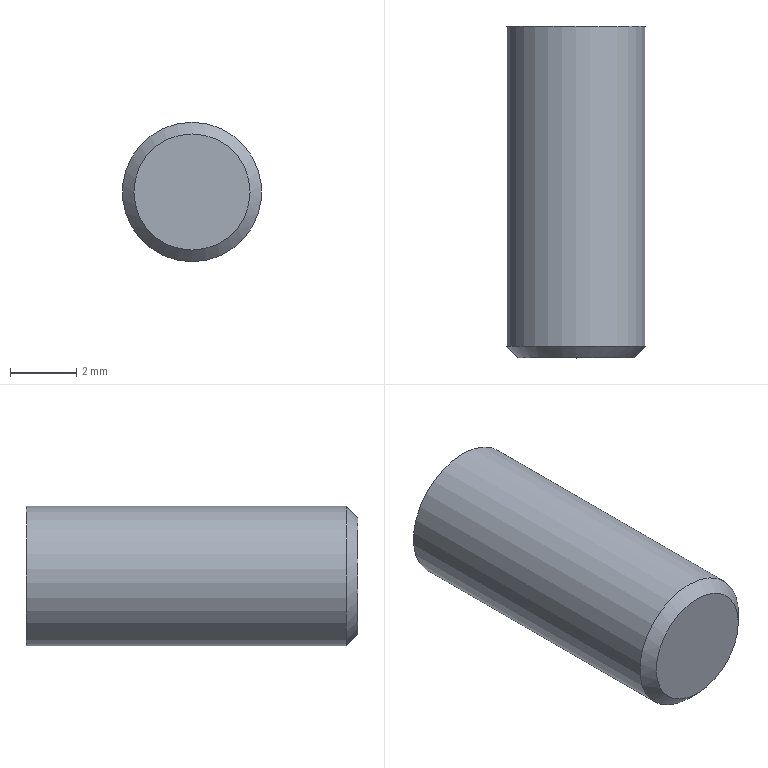Component | NX | 12_T77_2007_M5X10_FLAT_SET_SCREW | 1 solid | 11 faces | box 4.2 x 10 x 4.2 mm | volume 127 mm3 | plane 9 | cylinder 1 | cone 1 | commonest cylinder face diameters 4.2 x1
STEP:
#1=CARTESIAN_POINT('',(0.,0.,0.));
#2=DIRECTION('',(0.,0.,1.));
#3=DIRECTION('',(1.,0.,0.));
#4=AXIS2_PLACEMENT_3D('',#1,#2,#3);
#5=CARTESIAN_POINT('',(22.25,14.,74.278));
#6=VERTEX_POINT('',#5);
#7=CARTESIAN_POINT('',(22.25,14.,75.722));
#8=VERTEX_POINT('',#7);
#9=CARTESIAN_POINT('',(22.25,14.,74.278));
#10=DIRECTION('',(0.,0.,1.));
#11=VECTOR('',#10,1.);
#12=LINE('',#9,#11);
#13=CARTESIAN_POINT('',(21.,14.,75.));
#14=DIRECTION('',(0.,1.,0.));
#15=DIRECTION('',(0.,0.,-1.));
#16=AXIS2_PLACEMENT_3D('',#13,#14,#15);
#17=PLANE('',#16);
#18=CARTESIAN_POINT('',(0.7217,-1.25));
#19=DIRECTION('',(-1.,0.));
#20=VECTOR('',#19,1.);
#21=LINE('',#18,#20);
#22=(GEOMETRIC_REPRESENTATION_CONTEXT(2)PARAMETRIC_REPRESENTATION_CONTEXT()REPRESENTATION_CONTEXT('',''));
#23=DEFINITIONAL_REPRESENTATION('',(#21),#22);
#24=PCURVE('',#17,#23);
#25=CARTESIAN_POINT('',(22.25,12.,74.278));
#26=DIRECTION('',(-1.,0.,0.));
#27=DIRECTION('',(0.,0.,1.));
#28=AXIS2_PLACEMENT_3D('',#25,#26,#27);
#29=PLANE('',#28);
#30=CARTESIAN_POINT('',(0.,2.));
#31=DIRECTION('',(1.,0.));
#32=VECTOR('',#31,1.);
#33=LINE('',#30,#32);
#34=(GEOMETRIC_REPRESENTATION_CONTEXT(2)PARAMETRIC_REPRESENTATION_CONTEXT()REPRESENTATION_CONTEXT('',''));
#35=DEFINITIONAL_REPRESENTATION('',(#33),#34);
#36=PCURVE('',#29,#35);
#37=SURFACE_CURVE('',#12,(#24,#36),.PCURVE_S1.);
#38=EDGE_CURVE('',#6,#8,#37,.T.);
#39=ORIENTED_EDGE('',*,*,#38,.T.);
#40=CARTESIAN_POINT('',(21.,14.,76.443));
#41=VERTEX_POINT('',#40);
#42=CARTESIAN_POINT('',(22.25,14.,75.722));
#43=DIRECTION('',(-0.866,0.,0.5));
#44=VECTOR('',#43,1.);
#45=LINE('',#42,#44);
#46=CARTESIAN_POINT('',(-0.7217,-1.25));
#47=DIRECTION('',(-0.5,0.866));
#48=VECTOR('',#47,1.);
#49=LINE('',#46,#48);
#50=(GEOMETRIC_REPRESENTATION_CONTEXT(2)PARAMETRIC_REPRESENTATION_CONTEXT()REPRESENTATION_CONTEXT('',''));
#51=DEFINITIONAL_REPRESENTATION('',(#49),#50);
#52=PCURVE('',#17,#51);
#53=CARTESIAN_POINT('',(22.25,12.,75.722));
#54=DIRECTION('',(-0.5,0.,-0.866));
#55=DIRECTION('',(-0.866,0.,0.5));
#56=AXIS2_PLACEMENT_3D('',#53,#54,#55);
#57=PLANE('',#56);
#58=CARTESIAN_POINT('',(0.,2.));
#59=DIRECTION('',(1.,0.));
#60=VECTOR('',#59,1.);
#61=LINE('',#58,#60);
#62=(GEOMETRIC_REPRESENTATION_CONTEXT(2)PARAMETRIC_REPRESENTATION_CONTEXT()REPRESENTATION_CONTEXT('',''));
#63=DEFINITIONAL_REPRESENTATION('',(#61),#62);
#64=PCURVE('',#57,#63);
#65=SURFACE_CURVE('',#45,(#52,#64),.PCURVE_S1.);
#66=EDGE_CURVE('',#8,#41,#65,.T.);
#67=ORIENTED_EDGE('',*,*,#66,.T.);
#68=CARTESIAN_POINT('',(19.75,14.,75.722));
#69=VERTEX_POINT('',#68);
#70=CARTESIAN_POINT('',(21.,14.,76.443));
#71=DIRECTION('',(-0.866,0.,-0.5));
#72=VECTOR('',#71,1.);
#73=LINE('',#70,#72);
#74=CARTESIAN_POINT('',(-1.443,0.));
#75=DIRECTION('',(0.5,0.866));
#76=VECTOR('',#75,1.);
#77=LINE('',#74,#76);
#78=(GEOMETRIC_REPRESENTATION_CONTEXT(2)PARAMETRIC_REPRESENTATION_CONTEXT()REPRESENTATION_CONTEXT('',''));
#79=DEFINITIONAL_REPRESENTATION('',(#77),#78);
#80=PCURVE('',#17,#79);
#81=CARTESIAN_POINT('',(21.,12.,76.443));
#82=DIRECTION('',(0.5,0.,-0.866));
#83=DIRECTION('',(-0.866,0.,-0.5));
#84=AXIS2_PLACEMENT_3D('',#81,#82,#83);
#85=PLANE('',#84);
#86=CARTESIAN_POINT('',(0.,2.));
#87=DIRECTION('',(1.,0.));
#88=VECTOR('',#87,1.);
#89=LINE('',#86,#88);
#90=(GEOMETRIC_REPRESENTATION_CONTEXT(2)PARAMETRIC_REPRESENTATION_CONTEXT()REPRESENTATION_CONTEXT('',''));
#91=DEFINITIONAL_REPRESENTATION('',(#89),#90);
#92=PCURVE('',#85,#91);
#93=SURFACE_CURVE('',#73,(#80,#92),.PCURVE_S1.);
#94=EDGE_CURVE('',#41,#69,#93,.T.);
#95=ORIENTED_EDGE('',*,*,#94,.T.);
#96=CARTESIAN_POINT('',(19.75,14.,74.278));
#97=VERTEX_POINT('',#96);
#98=CARTESIAN_POINT('',(19.75,14.,75.722));
#99=DIRECTION('',(0.,0.,-1.));
#100=VECTOR('',#99,1.);
#101=LINE('',#98,#100);
#102=CARTESIAN_POINT('',(-0.7217,1.25));
#103=DIRECTION('',(1.,0.));
#104=VECTOR('',#103,1.);
#105=LINE('',#102,#104);
#106=(GEOMETRIC_REPRESENTATION_CONTEXT(2)PARAMETRIC_REPRESENTATION_CONTEXT()REPRESENTATION_CONTEXT('',''));
#107=DEFINITIONAL_REPRESENTATION('',(#105),#106);
#108=PCURVE('',#17,#107);
#109=CARTESIAN_POINT('',(19.75,12.,75.722));
#110=DIRECTION('',(1.,0.,0.));
#111=DIRECTION('',(0.,0.,-1.));
#112=AXIS2_PLACEMENT_3D('',#109,#110,#111);
#113=PLANE('',#112);
#114=CARTESIAN_POINT('',(0.,2.));
#115=DIRECTION('',(1.,0.));
#116=VECTOR('',#115,1.);
#117=LINE('',#114,#116);
#118=(GEOMETRIC_REPRESENTATION_CONTEXT(2)PARAMETRIC_REPRESENTATION_CONTEXT()REPRESENTATION_CONTEXT('',''));
#119=DEFINITIONAL_REPRESENTATION('',(#117),#118);
#120=PCURVE('',#113,#119);
#121=SURFACE_CURVE('',#101,(#108,#120),.PCURVE_S1.);
#122=EDGE_CURVE('',#69,#97,#121,.T.);
#123=ORIENTED_EDGE('',*,*,#122,.T.);
#124=CARTESIAN_POINT('',(21.,14.,73.557));
#125=VERTEX_POINT('',#124);
#126=CARTESIAN_POINT('',(19.75,14.,74.278));
#127=DIRECTION('',(0.866,-0.,-0.5));
#128=VECTOR('',#127,1.);
#129=LINE('',#126,#128);
#130=CARTESIAN_POINT('',(0.7217,1.25));
#131=DIRECTION('',(0.5,-0.866));
#132=VECTOR('',#131,1.);
#133=LINE('',#130,#132);
#134=(GEOMETRIC_REPRESENTATION_CONTEXT(2)PARAMETRIC_REPRESENTATION_CONTEXT()REPRESENTATION_CONTEXT('',''));
#135=DEFINITIONAL_REPRESENTATION('',(#133),#134);
#136=PCURVE('',#17,#135);
#137=CARTESIAN_POINT('',(19.75,12.,74.278));
#138=DIRECTION('',(0.5,0.,0.866));
#139=DIRECTION('',(0.866,0.,-0.5));
#140=AXIS2_PLACEMENT_3D('',#137,#138,#139);
#141=PLANE('',#140);
#142=CARTESIAN_POINT('',(0.,2.));
#143=DIRECTION('',(1.,-0.));
#144=VECTOR('',#143,1.);
#145=LINE('',#142,#144);
#146=(GEOMETRIC_REPRESENTATION_CONTEXT(2)PARAMETRIC_REPRESENTATION_CONTEXT()REPRESENTATION_CONTEXT('',''));
#147=DEFINITIONAL_REPRESENTATION('',(#145),#146);
#148=PCURVE('',#141,#147);
#149=SURFACE_CURVE('',#129,(#136,#148),.PCURVE_S1.);
#150=EDGE_CURVE('',#97,#125,#149,.T.);
#151=ORIENTED_EDGE('',*,*,#150,.T.);
#152=CARTESIAN_POINT('',(21.,14.,73.557));
#153=DIRECTION('',(0.866,-0.,0.5));
#154=VECTOR('',#153,1.);
#155=LINE('',#152,#154);
#156=CARTESIAN_POINT('',(1.443,0.));
#157=DIRECTION('',(-0.5,-0.866));
#158=VECTOR('',#157,1.);
#159=LINE('',#156,#158);
#160=(GEOMETRIC_REPRESENTATION_CONTEXT(2)PARAMETRIC_REPRESENTATION_CONTEXT()REPRESENTATION_CONTEXT('',''));
#161=DEFINITIONAL_REPRESENTATION('',(#159),#160);
#162=PCURVE('',#17,#161);
#163=CARTESIAN_POINT('',(21.,12.,73.557));
#164=DIRECTION('',(-0.5,0.,0.866));
#165=DIRECTION('',(0.866,0.,0.5));
#166=AXIS2_PLACEMENT_3D('',#163,#164,#165);
#167=PLANE('',#166);
#168=CARTESIAN_POINT('',(0.,2.));
#169=DIRECTION('',(1.,-0.));
#170=VECTOR('',#169,1.);
#171=LINE('',#168,#170);
#172=(GEOMETRIC_REPRESENTATION_CONTEXT(2)PARAMETRIC_REPRESENTATION_CONTEXT()REPRESENTATION_CONTEXT('',''));
#173=DEFINITIONAL_REPRESENTATION('',(#171),#172);
#174=PCURVE('',#167,#173);
#175=SURFACE_CURVE('',#155,(#162,#174),.PCURVE_S1.);
#176=EDGE_CURVE('',#125,#6,#175,.T.);
#177=ORIENTED_EDGE('',*,*,#176,.T.);
#178=EDGE_LOOP('',(#39,#67,#95,#123,#151,#177));
#179=FACE_BOUND('',#178,.T.);
#180=CARTESIAN_POINT('',(21.,14.,77.1));
#181=VERTEX_POINT('',#180);
#182=CARTESIAN_POINT('',(21.,14.,75.));
#183=DIRECTION('',(0.,1.,0.));
#184=DIRECTION('',(0.,-0.,1.));
#185=AXIS2_PLACEMENT_3D('',#182,#183,#184);
#186=CIRCLE('',#185,2.1);
#187=CARTESIAN_POINT('',(0.,0.));
#188=DIRECTION('',(-1.,0.));
#189=AXIS2_PLACEMENT_2D('',#187,#188);
#190=CIRCLE('',#189,2.1);
#191=(GEOMETRIC_REPRESENTATION_CONTEXT(2)PARAMETRIC_REPRESENTATION_CONTEXT()REPRESENTATION_CONTEXT('',''));
#192=DEFINITIONAL_REPRESENTATION('',(#190),#191);
#193=PCURVE('',#17,#192);
#194=CARTESIAN_POINT('',(21.,15.5,75.));
#195=DIRECTION('',(0.,-1.,0.));
#196=DIRECTION('',(0.,0.,-1.));
#197=AXIS2_PLACEMENT_3D('',#194,#195,#196);
#198=CYLINDRICAL_SURFACE('',#197,2.1);
#199=CARTESIAN_POINT('',(9.425,1.5));
#200=DIRECTION('',(-1.,0.));
#201=VECTOR('',#200,1.);
#202=LINE('',#199,#201);
#203=(GEOMETRIC_REPRESENTATION_CONTEXT(2)PARAMETRIC_REPRESENTATION_CONTEXT()REPRESENTATION_CONTEXT('',''));
#204=DEFINITIONAL_REPRESENTATION('',(#202),#203);
#205=PCURVE('',#198,#204);
#206=SURFACE_CURVE('',#186,(#193,#205),.PCURVE_S1.);
#207=EDGE_CURVE('',#181,#181,#206,.T.);
#208=ORIENTED_EDGE('',*,*,#207,.T.);
#209=EDGE_LOOP('',(#208));
#210=FACE_BOUND('',#209,.T.);
#211=ADVANCED_FACE('',(#179,#210),#17,.T.);
#212=ORIENTED_EDGE('',*,*,#66,.F.);
#213=CARTESIAN_POINT('',(22.25,12.,75.722));
#214=VERTEX_POINT('',#213);
#215=CARTESIAN_POINT('',(22.25,12.,75.722));
#216=DIRECTION('',(0.,1.,0.));
#217=VECTOR('',#216,1.);
#218=LINE('',#215,#217);
#219=CARTESIAN_POINT('',(0.,0.));
#220=DIRECTION('',(0.,1.));
#221=VECTOR('',#220,1.);
#222=LINE('',#219,#221);
#223=(GEOMETRIC_REPRESENTATION_CONTEXT(2)PARAMETRIC_REPRESENTATION_CONTEXT()REPRESENTATION_CONTEXT('',''));
#224=DEFINITIONAL_REPRESENTATION('',(#222),#223);
#225=PCURVE('',#57,#224);
#226=CARTESIAN_POINT('',(1.443,0.));
#227=DIRECTION('',(0.,1.));
#228=VECTOR('',#227,1.);
#229=LINE('',#226,#228);
#230=(GEOMETRIC_REPRESENTATION_CONTEXT(2)PARAMETRIC_REPRESENTATION_CONTEXT()REPRESENTATION_CONTEXT('',''));
#231=DEFINITIONAL_REPRESENTATION('',(#229),#230);
#232=PCURVE('',#29,#231);
#233=SURFACE_CURVE('',#218,(#225,#232),.PCURVE_S1.);
#234=EDGE_CURVE('',#214,#8,#233,.T.);
#235=ORIENTED_EDGE('',*,*,#234,.F.);
#236=CARTESIAN_POINT('',(21.,12.,76.443));
#237=VERTEX_POINT('',#236);
#238=CARTESIAN_POINT('',(22.25,12.,75.722));
#239=DIRECTION('',(-0.866,0.,0.5));
#240=VECTOR('',#239,1.);
#241=LINE('',#238,#240);
#242=CARTESIAN_POINT('',(0.,0.));
#243=DIRECTION('',(1.,0.));
#244=VECTOR('',#243,1.);
#245=LINE('',#242,#244);
#246=(GEOMETRIC_REPRESENTATION_CONTEXT(2)PARAMETRIC_REPRESENTATION_CONTEXT()REPRESENTATION_CONTEXT('',''));
#247=DEFINITIONAL_REPRESENTATION('',(#245),#246);
#248=PCURVE('',#57,#247);
#249=CARTESIAN_POINT('',(21.,12.,75.));
#250=DIRECTION('',(-0.,-1.,0.));
#251=DIRECTION('',(-1.,0.,0.));
#252=AXIS2_PLACEMENT_3D('',#249,#250,#251);
#253=PLANE('',#252);
#254=CARTESIAN_POINT('',(-1.25,-0.7217));
#255=DIRECTION('',(0.866,-0.5));
#256=VECTOR('',#255,1.);
#257=LINE('',#254,#256);
#258=(GEOMETRIC_REPRESENTATION_CONTEXT(2)PARAMETRIC_REPRESENTATION_CONTEXT()REPRESENTATION_CONTEXT('',''));
#259=DEFINITIONAL_REPRESENTATION('',(#257),#258);
#260=PCURVE('',#253,#259);
#261=SURFACE_CURVE('',#241,(#248,#260),.PCURVE_S1.);
#262=EDGE_CURVE('',#214,#237,#261,.T.);
#263=ORIENTED_EDGE('',*,*,#262,.T.);
#264=CARTESIAN_POINT('',(21.,12.,76.443));
#265=DIRECTION('',(0.,1.,0.));
#266=VECTOR('',#265,1.);
#267=LINE('',#264,#266);
#268=CARTESIAN_POINT('',(1.443,0.));
#269=DIRECTION('',(0.,1.));
#270=VECTOR('',#269,1.);
#271=LINE('',#268,#270);
#272=(GEOMETRIC_REPRESENTATION_CONTEXT(2)PARAMETRIC_REPRESENTATION_CONTEXT()REPRESENTATION_CONTEXT('',''));
#273=DEFINITIONAL_REPRESENTATION('',(#271),#272);
#274=PCURVE('',#57,#273);
#275=CARTESIAN_POINT('',(0.,0.));
#276=DIRECTION('',(0.,1.));
#277=VECTOR('',#276,1.);
#278=LINE('',#275,#277);
#279=(GEOMETRIC_REPRESENTATION_CONTEXT(2)PARAMETRIC_REPRESENTATION_CONTEXT()REPRESENTATION_CONTEXT('',''));
#280=DEFINITIONAL_REPRESENTATION('',(#278),#279);
#281=PCURVE('',#85,#280);
#282=SURFACE_CURVE('',#267,(#274,#281),.PCURVE_S1.);
#283=EDGE_CURVE('',#237,#41,#282,.T.);
#284=ORIENTED_EDGE('',*,*,#283,.T.);
#285=EDGE_LOOP('',(#212,#235,#263,#284));
#286=FACE_BOUND('',#285,.T.);
#287=ADVANCED_FACE('',(#286),#57,.T.);
#288=ORIENTED_EDGE('',*,*,#94,.F.);
#289=ORIENTED_EDGE('',*,*,#283,.F.);
#290=CARTESIAN_POINT('',(19.75,12.,75.722));
#291=VERTEX_POINT('',#290);
#292=CARTESIAN_POINT('',(21.,12.,76.443));
#293=DIRECTION('',(-0.866,0.,-0.5));
#294=VECTOR('',#293,1.);
#295=LINE('',#292,#294);
#296=CARTESIAN_POINT('',(0.,0.));
#297=DIRECTION('',(1.,0.));
#298=VECTOR('',#297,1.);
#299=LINE('',#296,#298);
#300=(GEOMETRIC_REPRESENTATION_CONTEXT(2)PARAMETRIC_REPRESENTATION_CONTEXT()REPRESENTATION_CONTEXT('',''));
#301=DEFINITIONAL_REPRESENTATION('',(#299),#300);
#302=PCURVE('',#85,#301);
#303=CARTESIAN_POINT('',(0.,-1.443));
#304=DIRECTION('',(0.866,0.5));
#305=VECTOR('',#304,1.);
#306=LINE('',#303,#305);
#307=(GEOMETRIC_REPRESENTATION_CONTEXT(2)PARAMETRIC_REPRESENTATION_CONTEXT()REPRESENTATION_CONTEXT('',''));
#308=DEFINITIONAL_REPRESENTATION('',(#306),#307);
#309=PCURVE('',#253,#308);
#310=SURFACE_CURVE('',#295,(#302,#309),.PCURVE_S1.);
#311=EDGE_CURVE('',#237,#291,#310,.T.);
#312=ORIENTED_EDGE('',*,*,#311,.T.);
#313=CARTESIAN_POINT('',(19.75,12.,75.722));
#314=DIRECTION('',(0.,1.,0.));
#315=VECTOR('',#314,1.);
#316=LINE('',#313,#315);
#317=CARTESIAN_POINT('',(1.443,0.));
#318=DIRECTION('',(0.,1.));
#319=VECTOR('',#318,1.);
#320=LINE('',#317,#319);
#321=(GEOMETRIC_REPRESENTATION_CONTEXT(2)PARAMETRIC_REPRESENTATION_CONTEXT()REPRESENTATION_CONTEXT('',''));
#322=DEFINITIONAL_REPRESENTATION('',(#320),#321);
#323=PCURVE('',#85,#322);
#324=CARTESIAN_POINT('',(0.,0.));
#325=DIRECTION('',(0.,1.));
#326=VECTOR('',#325,1.);
#327=LINE('',#324,#326);
#328=(GEOMETRIC_REPRESENTATION_CONTEXT(2)PARAMETRIC_REPRESENTATION_CONTEXT()REPRESENTATION_CONTEXT('',''));
#329=DEFINITIONAL_REPRESENTATION('',(#327),#328);
#330=PCURVE('',#113,#329);
#331=SURFACE_CURVE('',#316,(#323,#330),.PCURVE_S1.);
#332=EDGE_CURVE('',#291,#69,#331,.T.);
#333=ORIENTED_EDGE('',*,*,#332,.T.);
#334=EDGE_LOOP('',(#288,#289,#312,#333));
#335=FACE_BOUND('',#334,.T.);
#336=ADVANCED_FACE('',(#335),#85,.T.);
#337=ORIENTED_EDGE('',*,*,#122,.F.);
#338=ORIENTED_EDGE('',*,*,#332,.F.);
#339=CARTESIAN_POINT('',(19.75,12.,74.278));
#340=VERTEX_POINT('',#339);
#341=CARTESIAN_POINT('',(19.75,12.,75.722));
#342=DIRECTION('',(0.,0.,-1.));
#343=VECTOR('',#342,1.);
#344=LINE('',#341,#343);
#345=CARTESIAN_POINT('',(0.,0.));
#346=DIRECTION('',(1.,0.));
#347=VECTOR('',#346,1.);
#348=LINE('',#345,#347);
#349=(GEOMETRIC_REPRESENTATION_CONTEXT(2)PARAMETRIC_REPRESENTATION_CONTEXT()REPRESENTATION_CONTEXT('',''));
#350=DEFINITIONAL_REPRESENTATION('',(#348),#349);
#351=PCURVE('',#113,#350);
#352=CARTESIAN_POINT('',(1.25,-0.7217));
#353=DIRECTION('',(0.,1.));
#354=VECTOR('',#353,1.);
#355=LINE('',#352,#354);
#356=(GEOMETRIC_REPRESENTATION_CONTEXT(2)PARAMETRIC_REPRESENTATION_CONTEXT()REPRESENTATION_CONTEXT('',''));
#357=DEFINITIONAL_REPRESENTATION('',(#355),#356);
#358=PCURVE('',#253,#357);
#359=SURFACE_CURVE('',#344,(#351,#358),.PCURVE_S1.);
#360=EDGE_CURVE('',#291,#340,#359,.T.);
#361=ORIENTED_EDGE('',*,*,#360,.T.);
#362=CARTESIAN_POINT('',(19.75,12.,74.278));
#363=DIRECTION('',(0.,1.,0.));
#364=VECTOR('',#363,1.);
#365=LINE('',#362,#364);
#366=CARTESIAN_POINT('',(1.443,0.));
#367=DIRECTION('',(0.,1.));
#368=VECTOR('',#367,1.);
#369=LINE('',#366,#368);
#370=(GEOMETRIC_REPRESENTATION_CONTEXT(2)PARAMETRIC_REPRESENTATION_CONTEXT()REPRESENTATION_CONTEXT('',''));
#371=DEFINITIONAL_REPRESENTATION('',(#369),#370);
#372=PCURVE('',#113,#371);
#373=CARTESIAN_POINT('',(0.,0.));
#374=DIRECTION('',(0.,1.));
#375=VECTOR('',#374,1.);
#376=LINE('',#373,#375);
#377=(GEOMETRIC_REPRESENTATION_CONTEXT(2)PARAMETRIC_REPRESENTATION_CONTEXT()REPRESENTATION_CONTEXT('',''));
#378=DEFINITIONAL_REPRESENTATION('',(#376),#377);
#379=PCURVE('',#141,#378);
#380=SURFACE_CURVE('',#365,(#372,#379),.PCURVE_S1.);
#381=EDGE_CURVE('',#340,#97,#380,.T.);
#382=ORIENTED_EDGE('',*,*,#381,.T.);
#383=EDGE_LOOP('',(#337,#338,#361,#382));
#384=FACE_BOUND('',#383,.T.);
#385=ADVANCED_FACE('',(#384),#113,.T.);
#386=ORIENTED_EDGE('',*,*,#150,.F.);
#387=ORIENTED_EDGE('',*,*,#381,.F.);
#388=CARTESIAN_POINT('',(21.,12.,73.557));
#389=VERTEX_POINT('',#388);
#390=CARTESIAN_POINT('',(19.75,12.,74.278));
#391=DIRECTION('',(0.866,-0.,-0.5));
#392=VECTOR('',#391,1.);
#393=LINE('',#390,#392);
#394=CARTESIAN_POINT('',(0.,0.));
#395=DIRECTION('',(1.,-0.));
#396=VECTOR('',#395,1.);
#397=LINE('',#394,#396);
#398=(GEOMETRIC_REPRESENTATION_CONTEXT(2)PARAMETRIC_REPRESENTATION_CONTEXT()REPRESENTATION_CONTEXT('',''));
#399=DEFINITIONAL_REPRESENTATION('',(#397),#398);
#400=PCURVE('',#141,#399);
#401=CARTESIAN_POINT('',(1.25,0.7217));
#402=DIRECTION('',(-0.866,0.5));
#403=VECTOR('',#402,1.);
#404=LINE('',#401,#403);
#405=(GEOMETRIC_REPRESENTATION_CONTEXT(2)PARAMETRIC_REPRESENTATION_CONTEXT()REPRESENTATION_CONTEXT('',''));
#406=DEFINITIONAL_REPRESENTATION('',(#404),#405);
#407=PCURVE('',#253,#406);
#408=SURFACE_CURVE('',#393,(#400,#407),.PCURVE_S1.);
#409=EDGE_CURVE('',#340,#389,#408,.T.);
#410=ORIENTED_EDGE('',*,*,#409,.T.);
#411=CARTESIAN_POINT('',(21.,12.,73.557));
#412=DIRECTION('',(0.,1.,0.));
#413=VECTOR('',#412,1.);
#414=LINE('',#411,#413);
#415=CARTESIAN_POINT('',(1.443,0.));
#416=DIRECTION('',(0.,1.));
#417=VECTOR('',#416,1.);
#418=LINE('',#415,#417);
#419=(GEOMETRIC_REPRESENTATION_CONTEXT(2)PARAMETRIC_REPRESENTATION_CONTEXT()REPRESENTATION_CONTEXT('',''));
#420=DEFINITIONAL_REPRESENTATION('',(#418),#419);
#421=PCURVE('',#141,#420);
#422=CARTESIAN_POINT('',(0.,0.));
#423=DIRECTION('',(0.,1.));
#424=VECTOR('',#423,1.);
#425=LINE('',#422,#424);
#426=(GEOMETRIC_REPRESENTATION_CONTEXT(2)PARAMETRIC_REPRESENTATION_CONTEXT()REPRESENTATION_CONTEXT('',''));
#427=DEFINITIONAL_REPRESENTATION('',(#425),#426);
#428=PCURVE('',#167,#427);
#429=SURFACE_CURVE('',#414,(#421,#428),.PCURVE_S1.);
#430=EDGE_CURVE('',#389,#125,#429,.T.);
#431=ORIENTED_EDGE('',*,*,#430,.T.);
#432=EDGE_LOOP('',(#386,#387,#410,#431));
#433=FACE_BOUND('',#432,.T.);
#434=ADVANCED_FACE('',(#433),#141,.T.);
#435=ORIENTED_EDGE('',*,*,#176,.F.);
#436=ORIENTED_EDGE('',*,*,#430,.F.);
#437=CARTESIAN_POINT('',(22.25,12.,74.278));
#438=VERTEX_POINT('',#437);
#439=CARTESIAN_POINT('',(21.,12.,73.557));
#440=DIRECTION('',(0.866,-0.,0.5));
#441=VECTOR('',#440,1.);
#442=LINE('',#439,#441);
#443=CARTESIAN_POINT('',(0.,0.));
#444=DIRECTION('',(1.,-0.));
#445=VECTOR('',#444,1.);
#446=LINE('',#443,#445);
#447=(GEOMETRIC_REPRESENTATION_CONTEXT(2)PARAMETRIC_REPRESENTATION_CONTEXT()REPRESENTATION_CONTEXT('',''));
#448=DEFINITIONAL_REPRESENTATION('',(#446),#447);
#449=PCURVE('',#167,#448);
#450=CARTESIAN_POINT('',(0.,1.443));
#451=DIRECTION('',(-0.866,-0.5));
#452=VECTOR('',#451,1.);
#453=LINE('',#450,#452);
#454=(GEOMETRIC_REPRESENTATION_CONTEXT(2)PARAMETRIC_REPRESENTATION_CONTEXT()REPRESENTATION_CONTEXT('',''));
#455=DEFINITIONAL_REPRESENTATION('',(#453),#454);
#456=PCURVE('',#253,#455);
#457=SURFACE_CURVE('',#442,(#449,#456),.PCURVE_S1.);
#458=EDGE_CURVE('',#389,#438,#457,.T.);
#459=ORIENTED_EDGE('',*,*,#458,.T.);
#460=CARTESIAN_POINT('',(22.25,12.,74.278));
#461=DIRECTION('',(0.,1.,0.));
#462=VECTOR('',#461,1.);
#463=LINE('',#460,#462);
#464=CARTESIAN_POINT('',(1.443,0.));
#465=DIRECTION('',(0.,1.));
#466=VECTOR('',#465,1.);
#467=LINE('',#464,#466);
#468=(GEOMETRIC_REPRESENTATION_CONTEXT(2)PARAMETRIC_REPRESENTATION_CONTEXT()REPRESENTATION_CONTEXT('',''));
#469=DEFINITIONAL_REPRESENTATION('',(#467),#468);
#470=PCURVE('',#167,#469);
#471=CARTESIAN_POINT('',(0.,0.));
#472=DIRECTION('',(0.,1.));
#473=VECTOR('',#472,1.);
#474=LINE('',#471,#473);
#475=(GEOMETRIC_REPRESENTATION_CONTEXT(2)PARAMETRIC_REPRESENTATION_CONTEXT()REPRESENTATION_CONTEXT('',''));
#476=DEFINITIONAL_REPRESENTATION('',(#474),#475);
#477=PCURVE('',#29,#476);
#478=SURFACE_CURVE('',#463,(#470,#477),.PCURVE_S1.);
#479=EDGE_CURVE('',#438,#6,#478,.T.);
#480=ORIENTED_EDGE('',*,*,#479,.T.);
#481=EDGE_LOOP('',(#435,#436,#459,#480));
#482=FACE_BOUND('',#481,.T.);
#483=ADVANCED_FACE('',(#482),#167,.T.);
#484=ORIENTED_EDGE('',*,*,#38,.F.);
#485=ORIENTED_EDGE('',*,*,#479,.F.);
#486=CARTESIAN_POINT('',(22.25,12.,74.278));
#487=DIRECTION('',(0.,0.,1.));
#488=VECTOR('',#487,1.);
#489=LINE('',#486,#488);
#490=CARTESIAN_POINT('',(0.,0.));
#491=DIRECTION('',(1.,0.));
#492=VECTOR('',#491,1.);
#493=LINE('',#490,#492);
#494=(GEOMETRIC_REPRESENTATION_CONTEXT(2)PARAMETRIC_REPRESENTATION_CONTEXT()REPRESENTATION_CONTEXT('',''));
#495=DEFINITIONAL_REPRESENTATION('',(#493),#494);
#496=PCURVE('',#29,#495);
#497=CARTESIAN_POINT('',(-1.25,0.7217));
#498=DIRECTION('',(0.,-1.));
#499=VECTOR('',#498,1.);
#500=LINE('',#497,#499);
#501=(GEOMETRIC_REPRESENTATION_CONTEXT(2)PARAMETRIC_REPRESENTATION_CONTEXT()REPRESENTATION_CONTEXT('',''));
#502=DEFINITIONAL_REPRESENTATION('',(#500),#501);
#503=PCURVE('',#253,#502);
#504=SURFACE_CURVE('',#489,(#496,#503),.PCURVE_S1.);
#505=EDGE_CURVE('',#438,#214,#504,.T.);
#506=ORIENTED_EDGE('',*,*,#505,.T.);
#507=ORIENTED_EDGE('',*,*,#234,.T.);
#508=EDGE_LOOP('',(#484,#485,#506,#507));
#509=FACE_BOUND('',#508,.T.);
#510=ADVANCED_FACE('',(#509),#29,.T.);
#511=ORIENTED_EDGE('',*,*,#262,.F.);
#512=ORIENTED_EDGE('',*,*,#505,.F.);
#513=ORIENTED_EDGE('',*,*,#458,.F.);
#514=ORIENTED_EDGE('',*,*,#409,.F.);
#515=ORIENTED_EDGE('',*,*,#360,.F.);
#516=ORIENTED_EDGE('',*,*,#311,.F.);
#517=EDGE_LOOP('',(#511,#512,#513,#514,#515,#516));
#518=FACE_BOUND('',#517,.T.);
#519=ADVANCED_FACE('',(#518),#253,.F.);
#520=ORIENTED_EDGE('',*,*,#207,.F.);
#521=CARTESIAN_POINT('',(21.,4.35,77.1));
#522=VERTEX_POINT('',#521);
#523=CARTESIAN_POINT('',(21.,14.,77.1));
#524=CARTESIAN_POINT('',(21.,4.35,77.1));
#525=B_SPLINE_CURVE_WITH_KNOTS('',1,(#523,#524),.UNSPECIFIED.,.F.,.F.,(2,2),(1.5,11.15),.PIECEWISE_BEZIER_KNOTS.);
#526=CARTESIAN_POINT('',(9.425,0.));
#527=DIRECTION('',(0.,1.));
#528=VECTOR('',#527,1.);
#529=LINE('',#526,#528);
#530=(GEOMETRIC_REPRESENTATION_CONTEXT(2)PARAMETRIC_REPRESENTATION_CONTEXT()REPRESENTATION_CONTEXT('',''));
#531=DEFINITIONAL_REPRESENTATION('',(#529),#530);
#532=PCURVE('',#198,#531);
#533=CARTESIAN_POINT('',(3.142,0.));
#534=DIRECTION('',(0.,1.));
#535=VECTOR('',#534,1.);
#536=LINE('',#533,#535);
#537=(GEOMETRIC_REPRESENTATION_CONTEXT(2)PARAMETRIC_REPRESENTATION_CONTEXT()REPRESENTATION_CONTEXT('',''));
#538=DEFINITIONAL_REPRESENTATION('',(#536),#537);
#539=PCURVE('',#198,#538);
#540=SEAM_CURVE('',#525,(#532,#539),.PCURVE_S1.);
#541=EDGE_CURVE('',#181,#522,#540,.T.);
#542=ORIENTED_EDGE('',*,*,#541,.T.);
#543=CARTESIAN_POINT('',(21.,4.35,75.));
#544=DIRECTION('',(0.,-1.,-0.));
#545=DIRECTION('',(0.,-0.,1.));
#546=AXIS2_PLACEMENT_3D('',#543,#544,#545);
#547=CIRCLE('',#546,2.1);
#548=CARTESIAN_POINT('',(3.142,11.15));
#549=DIRECTION('',(1.,0.));
#550=VECTOR('',#549,1.);
#551=LINE('',#548,#550);
#552=(GEOMETRIC_REPRESENTATION_CONTEXT(2)PARAMETRIC_REPRESENTATION_CONTEXT()REPRESENTATION_CONTEXT('',''));
#553=DEFINITIONAL_REPRESENTATION('',(#551),#552);
#554=PCURVE('',#198,#553);
#555=CARTESIAN_POINT('',(21.,4.75,75.));
#556=DIRECTION('',(0.,1.,0.));
#557=DIRECTION('',(0.,0.,-1.));
#558=AXIS2_PLACEMENT_3D('',#555,#556,#557);
#559=CONICAL_SURFACE('',#558,2.5,0.7854);
#560=CARTESIAN_POINT('',(9.425,-0.4));
#561=DIRECTION('',(-1.,0.));
#562=VECTOR('',#561,1.);
#563=LINE('',#560,#562);
#564=(GEOMETRIC_REPRESENTATION_CONTEXT(2)PARAMETRIC_REPRESENTATION_CONTEXT()REPRESENTATION_CONTEXT('',''));
#565=DEFINITIONAL_REPRESENTATION('',(#563),#564);
#566=PCURVE('',#559,#565);
#567=SURFACE_CURVE('',#547,(#554,#566),.PCURVE_S1.);
#568=EDGE_CURVE('',#522,#522,#567,.T.);
#569=ORIENTED_EDGE('',*,*,#568,.F.);
#570=ORIENTED_EDGE('',*,*,#541,.F.);
#571=EDGE_LOOP('',(#520,#542,#569,#570));
#572=FACE_BOUND('',#571,.T.);
#573=ADVANCED_FACE('',(#572),#198,.T.);
#574=CARTESIAN_POINT('',(21.,4.,76.75));
#575=VERTEX_POINT('',#574);
#576=CARTESIAN_POINT('',(21.,4.,75.));
#577=DIRECTION('',(0.,1.,0.));
#578=DIRECTION('',(0.,-0.,1.));
#579=AXIS2_PLACEMENT_3D('',#576,#577,#578);
#580=CIRCLE('',#579,1.75);
#581=CARTESIAN_POINT('',(21.,4.,76.75));
#582=DIRECTION('',(0.,-1.,-0.));
#583=DIRECTION('',(0.,-0.,1.));
#584=AXIS2_PLACEMENT_3D('',#581,#582,#583);
#585=PLANE('',#584);
#586=CARTESIAN_POINT('',(-0.,0.));
#587=CARTESIAN_POINT('',(-0.,-3.031));
#588=CARTESIAN_POINT('',(-2.625,-1.516));
#589=CARTESIAN_POINT('',(-5.25,-0.));
#590=CARTESIAN_POINT('',(-2.625,1.516));
#591=CARTESIAN_POINT('',(-0.,3.031));
#592=CARTESIAN_POINT('',(-0.,0.));
#593=(BOUNDED_CURVE()B_SPLINE_CURVE(2,(#586,#587,#588,#589,#590,#591,#592),.UNSPECIFIED.,.T.,.F.)B_SPLINE_CURVE_WITH_KNOTS((1,2,2,2,2,1),(-2.094,0.,2.094,4.189,6.283,8.378),.UNSPECIFIED.)CURVE()GEOMETRIC_REPRESENTATION_ITEM()RATIONAL_B_SPLINE_CURVE((1.,0.5,1.,0.5,1.,0.5,1.))REPRESENTATION_ITEM(''));
#594=(GEOMETRIC_REPRESENTATION_CONTEXT(2)PARAMETRIC_REPRESENTATION_CONTEXT()REPRESENTATION_CONTEXT('',''));
#595=DEFINITIONAL_REPRESENTATION('',(#593),#594);
#596=PCURVE('',#585,#595);
#597=CARTESIAN_POINT('',(3.142,-0.75));
#598=DIRECTION('',(1.,0.));
#599=VECTOR('',#598,1.);
#600=LINE('',#597,#599);
#601=(GEOMETRIC_REPRESENTATION_CONTEXT(2)PARAMETRIC_REPRESENTATION_CONTEXT()REPRESENTATION_CONTEXT('',''));
#602=DEFINITIONAL_REPRESENTATION('',(#600),#601);
#603=PCURVE('',#559,#602);
#604=SURFACE_CURVE('',#580,(#596,#603),.PCURVE_S1.);
#605=EDGE_CURVE('',#575,#575,#604,.T.);
#606=ORIENTED_EDGE('',*,*,#605,.F.);
#607=EDGE_LOOP('',(#606));
#608=FACE_BOUND('',#607,.T.);
#609=ADVANCED_FACE('',(#608),#585,.T.);
#610=ORIENTED_EDGE('',*,*,#605,.T.);
#611=CARTESIAN_POINT('',(21.,4.,76.75));
#612=CARTESIAN_POINT('',(21.,4.35,77.1));
#613=B_SPLINE_CURVE_WITH_KNOTS('',1,(#611,#612),.UNSPECIFIED.,.F.,.F.,(2,2),(-1.061,-0.5657),.PIECEWISE_BEZIER_KNOTS.);
#614=CARTESIAN_POINT('',(9.425,0.));
#615=DIRECTION('',(0.,1.));
#616=VECTOR('',#615,1.);
#617=LINE('',#614,#616);
#618=(GEOMETRIC_REPRESENTATION_CONTEXT(2)PARAMETRIC_REPRESENTATION_CONTEXT()REPRESENTATION_CONTEXT('',''));
#619=DEFINITIONAL_REPRESENTATION('',(#617),#618);
#620=PCURVE('',#559,#619);
#621=CARTESIAN_POINT('',(3.142,0.));
#622=DIRECTION('',(0.,1.));
#623=VECTOR('',#622,1.);
#624=LINE('',#621,#623);
#625=(GEOMETRIC_REPRESENTATION_CONTEXT(2)PARAMETRIC_REPRESENTATION_CONTEXT()REPRESENTATION_CONTEXT('',''));
#626=DEFINITIONAL_REPRESENTATION('',(#624),#625);
#627=PCURVE('',#559,#626);
#628=SEAM_CURVE('',#613,(#620,#627),.PCURVE_S1.);
#629=EDGE_CURVE('',#575,#522,#628,.T.);
#630=ORIENTED_EDGE('',*,*,#629,.T.);
#631=ORIENTED_EDGE('',*,*,#568,.T.);
#632=ORIENTED_EDGE('',*,*,#629,.F.);
#633=EDGE_LOOP('',(#610,#630,#631,#632));
#634=FACE_BOUND('',#633,.T.);
#635=ADVANCED_FACE('',(#634),#559,.T.);
#636=CLOSED_SHELL('',(#211,#287,#336,#385,#434,#483,#510,#519,#573,#609,#635));
#637=MANIFOLD_SOLID_BREP('',#636);
#638=(LENGTH_UNIT()NAMED_UNIT(*)SI_UNIT(.MILLI.,.METRE.));
#639=UNCERTAINTY_MEASURE_WITH_UNIT(LENGTH_MEASURE(0.000002),#638,'','');
#640=(NAMED_UNIT(*)PLANE_ANGLE_UNIT()SI_UNIT($,.RADIAN.));
#641=(NAMED_UNIT(*)SI_UNIT($,.STERADIAN.)SOLID_ANGLE_UNIT());
#642=(GEOMETRIC_REPRESENTATION_CONTEXT(3)GLOBAL_UNCERTAINTY_ASSIGNED_CONTEXT((#639))GLOBAL_UNIT_ASSIGNED_CONTEXT((#638,#640,#641))REPRESENTATION_CONTEXT('',''));
#643=ADVANCED_BREP_SHAPE_REPRESENTATION('',(#4,#637),#642);